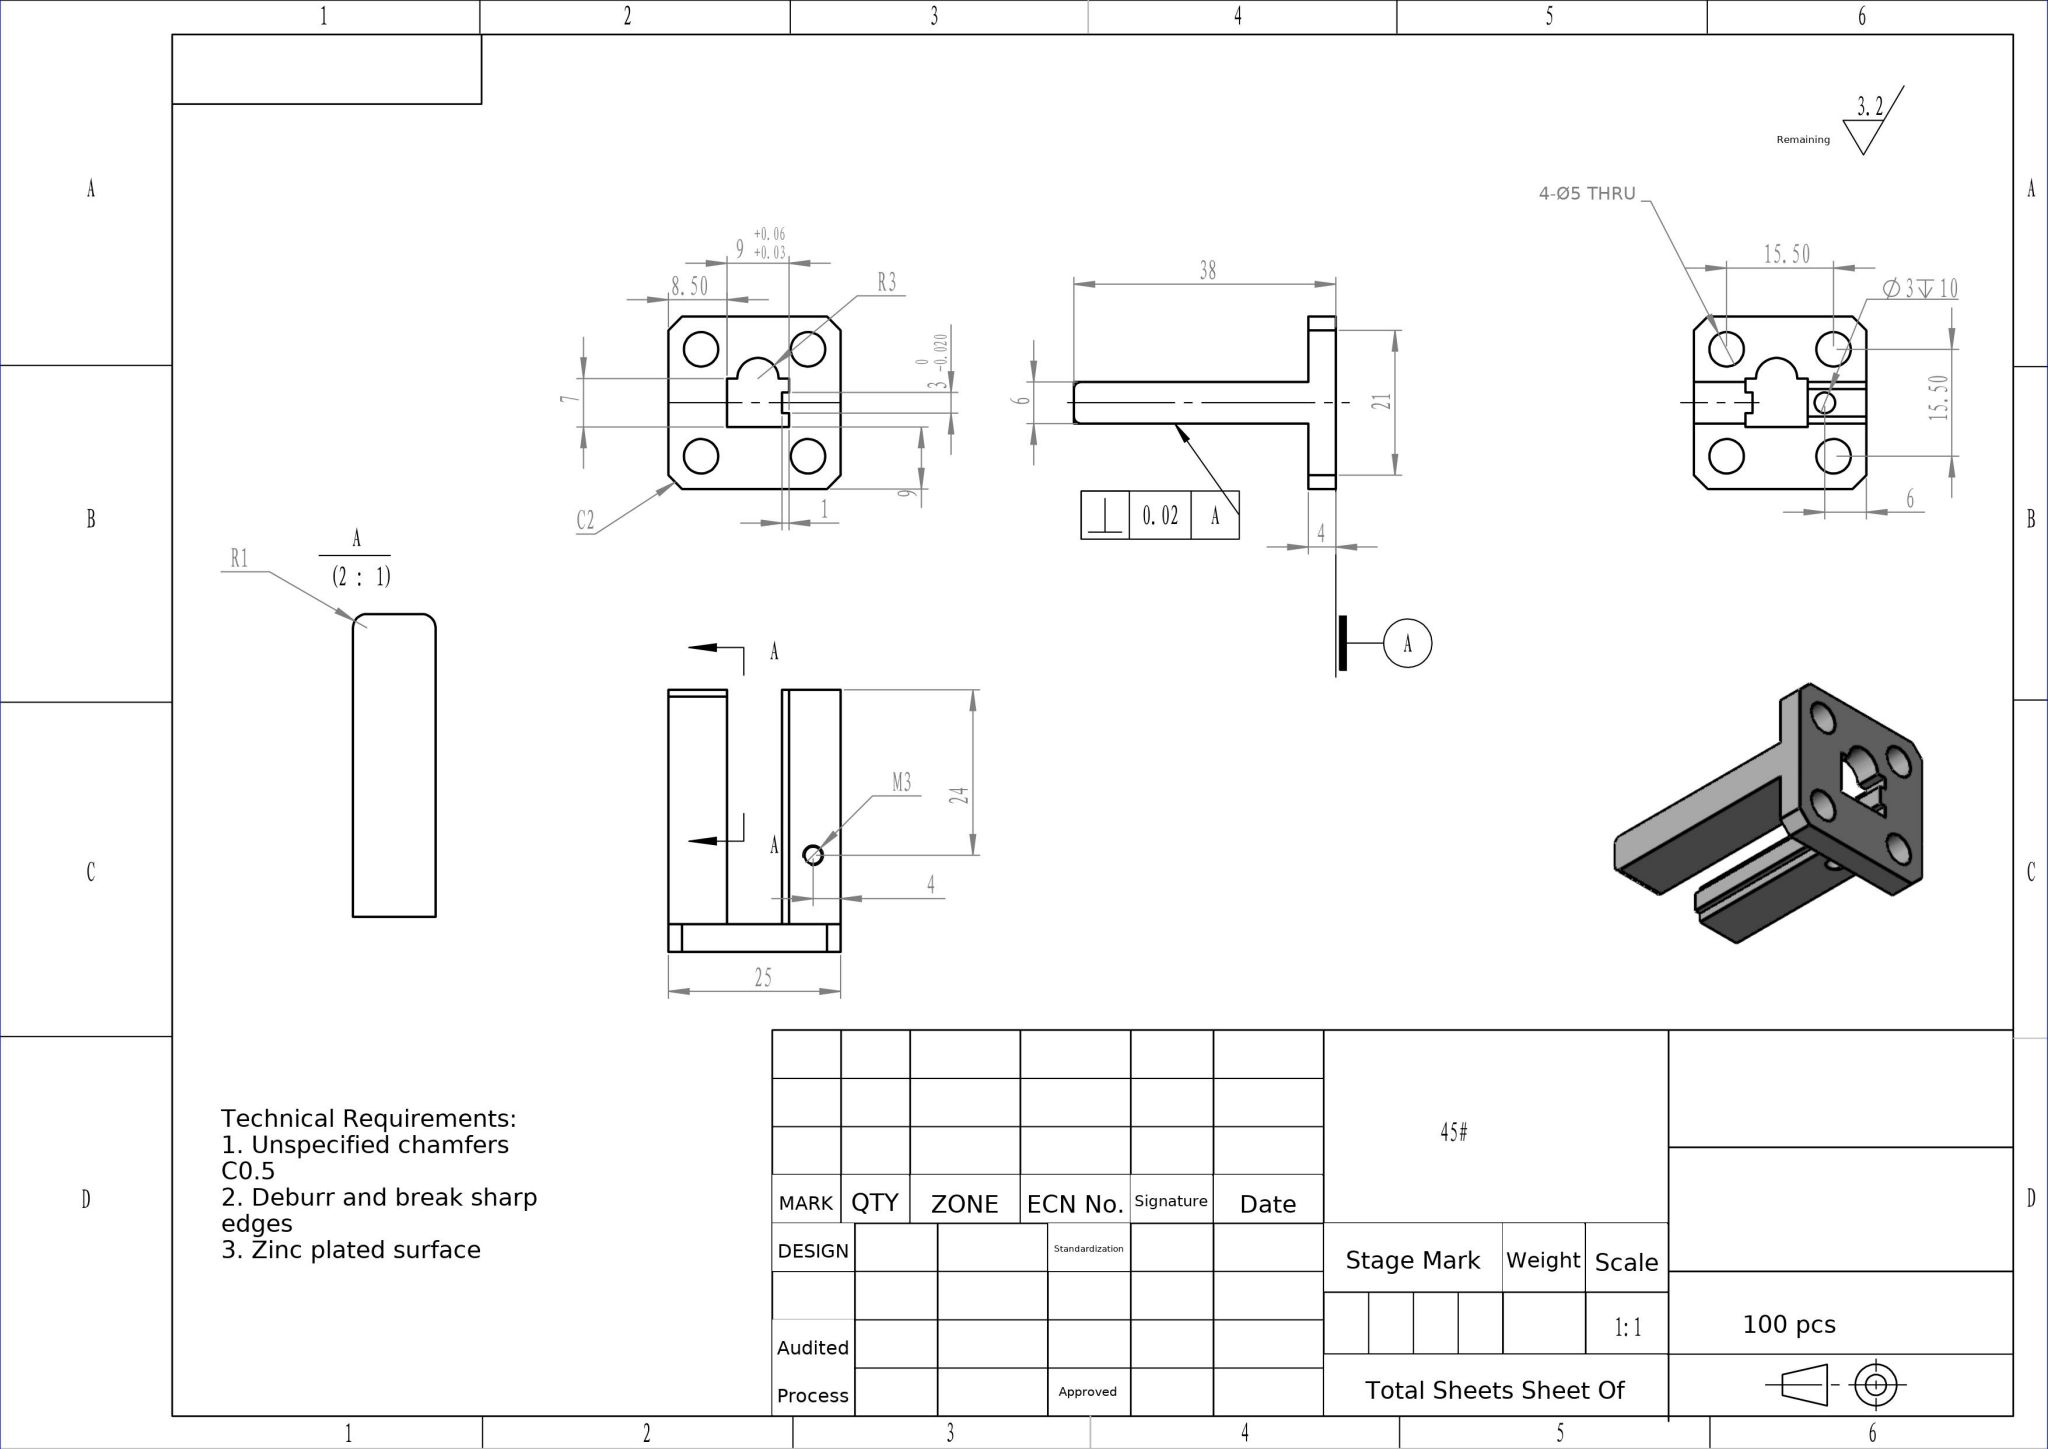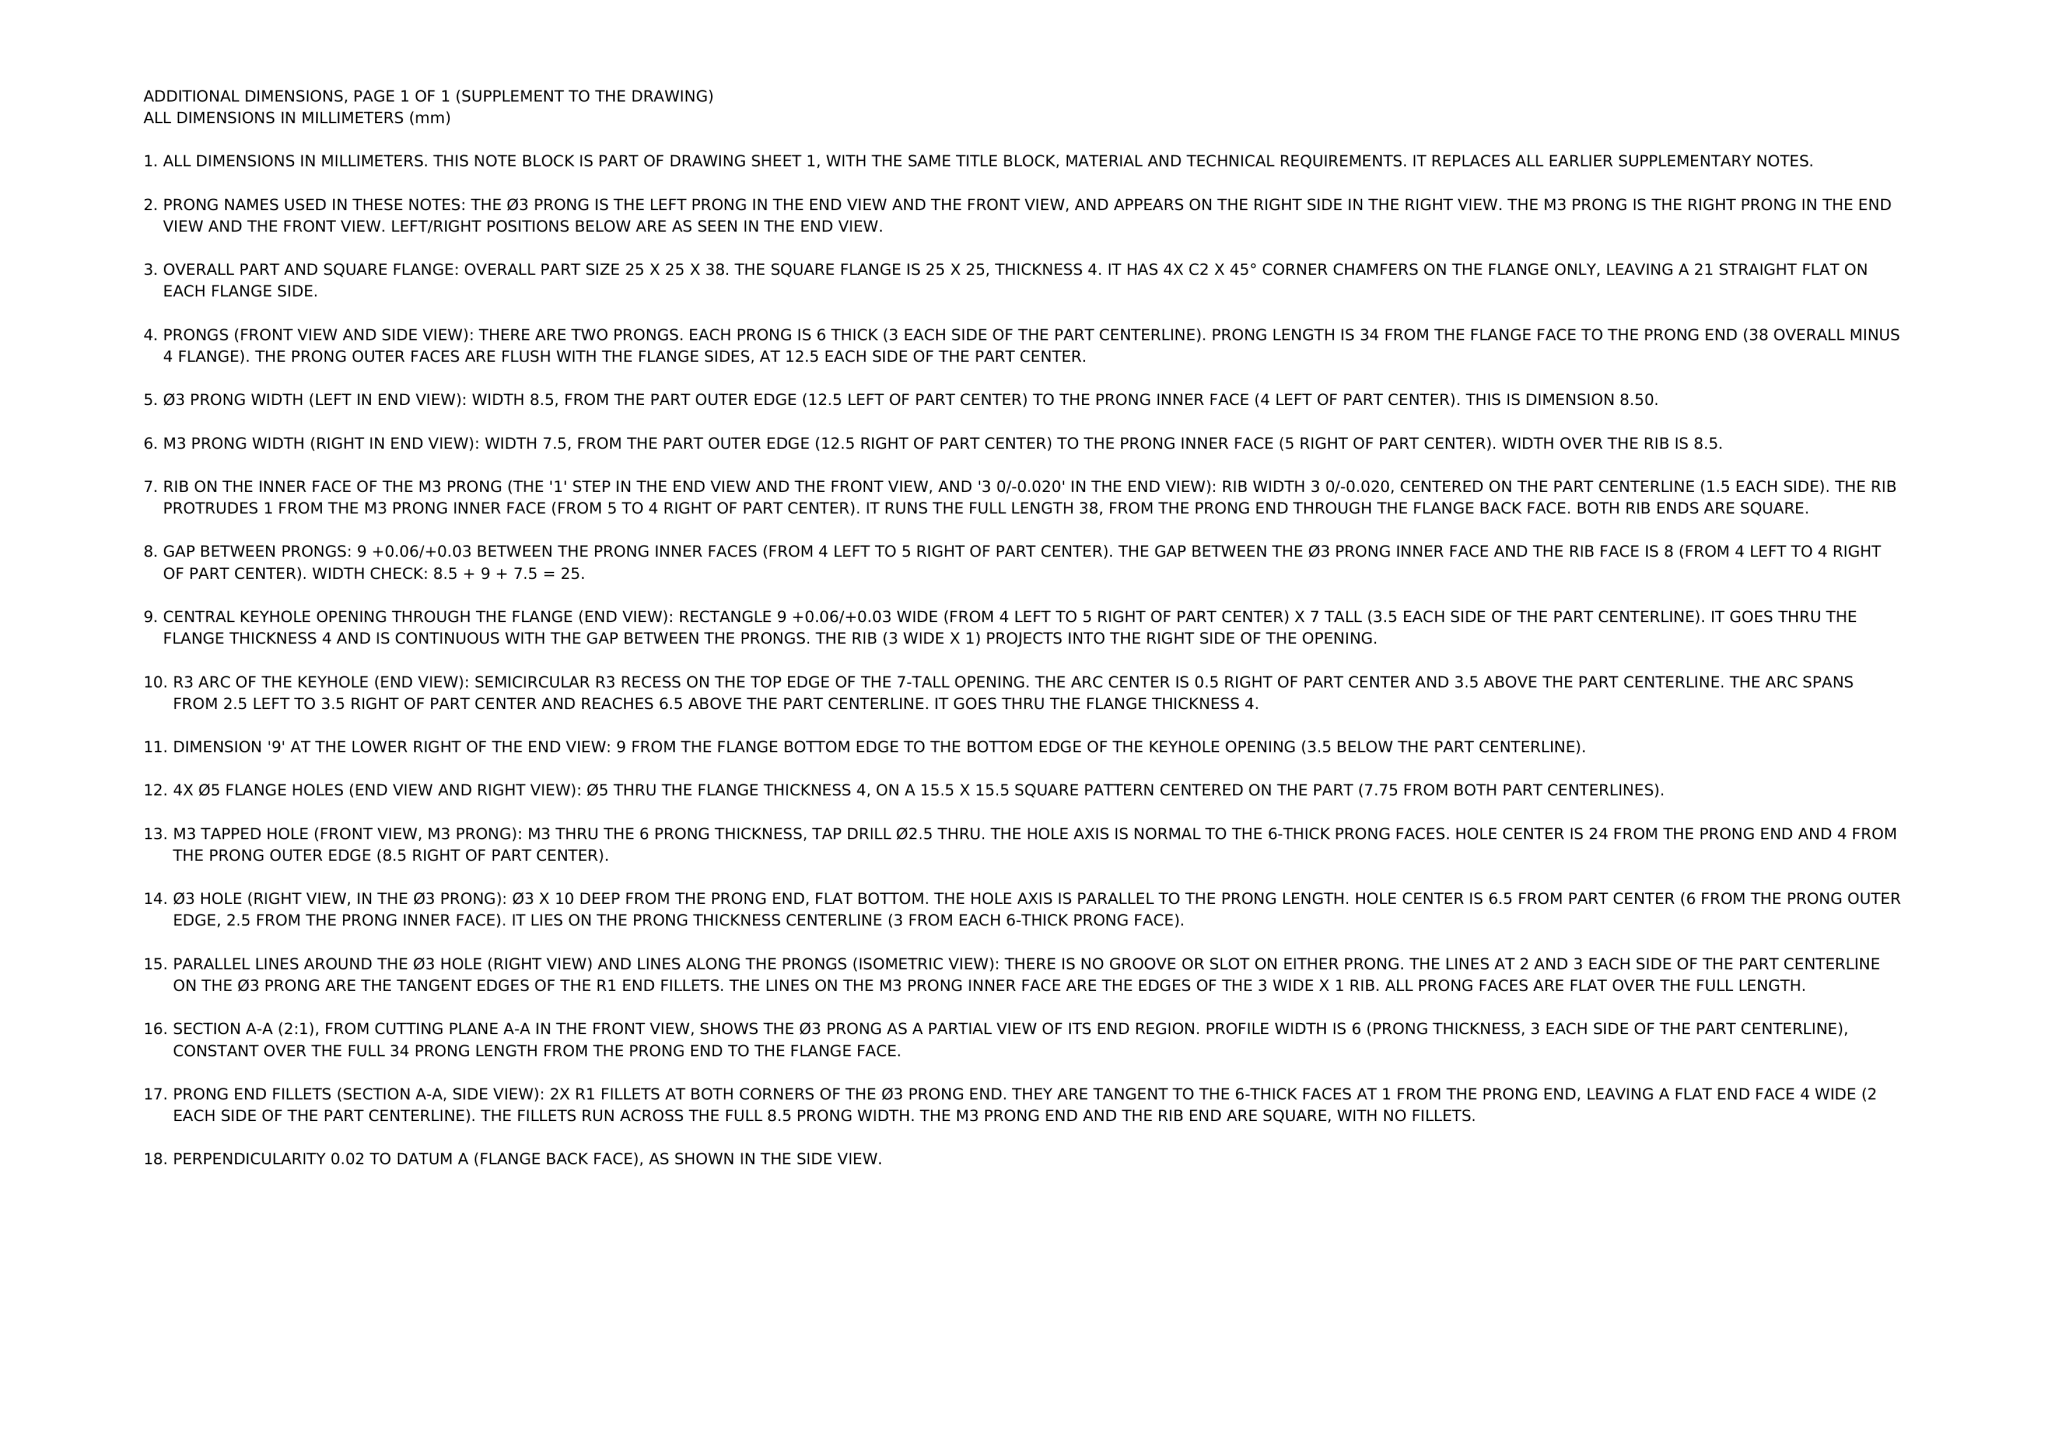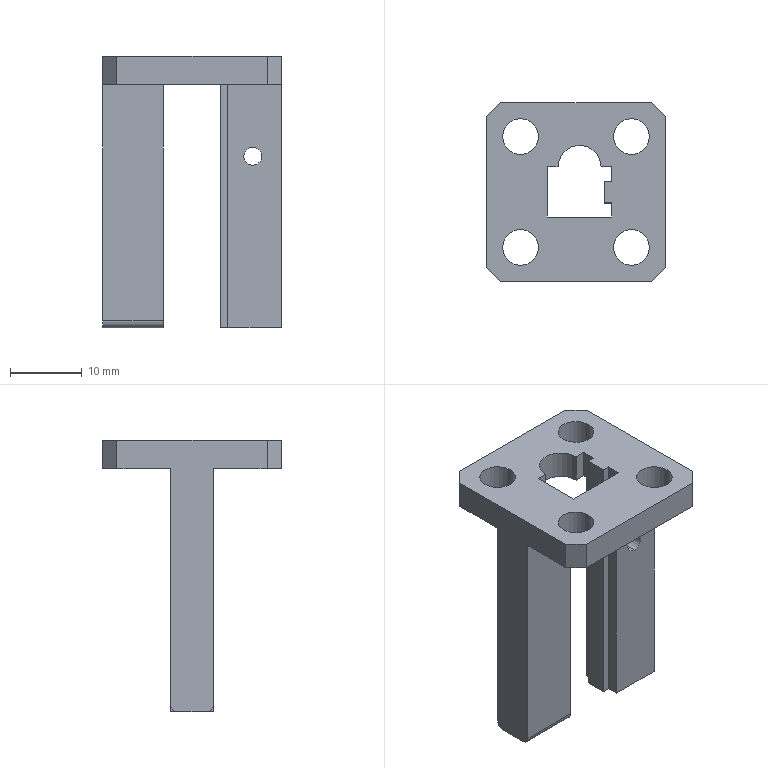Part | NX | mm | 1 solid | 42 faces | box 25 x 25 x 38 mm | volume 5120 mm3 | plane 27 | cylinder 15 | commonest cylinder face diameters 5 x8 3 x2 2.5 x2 2 x2 6 x1